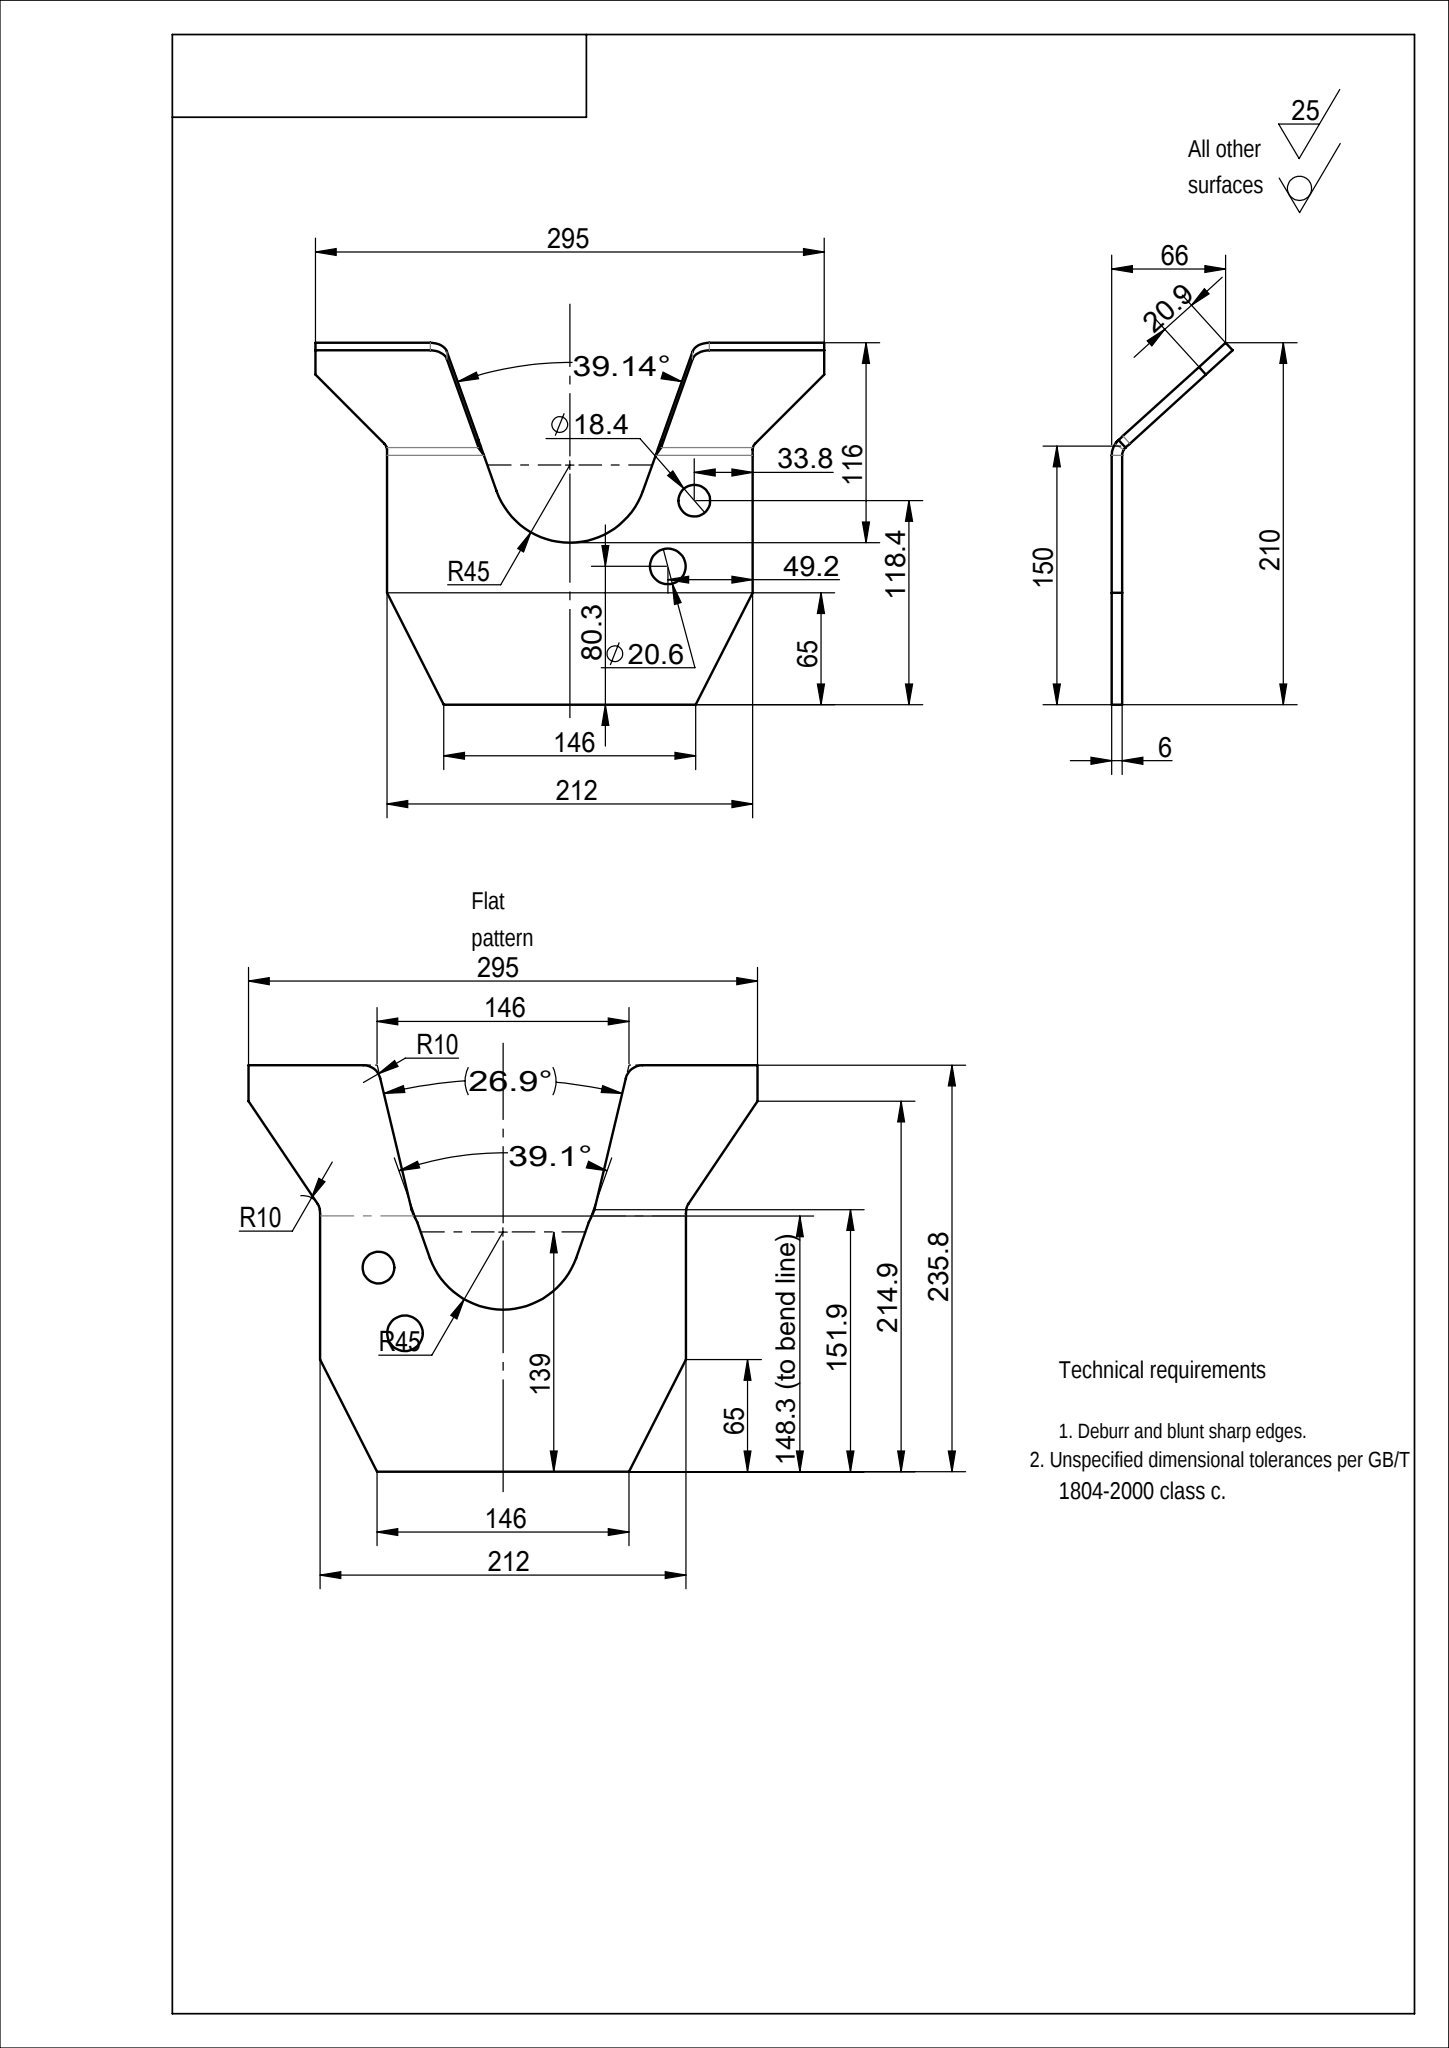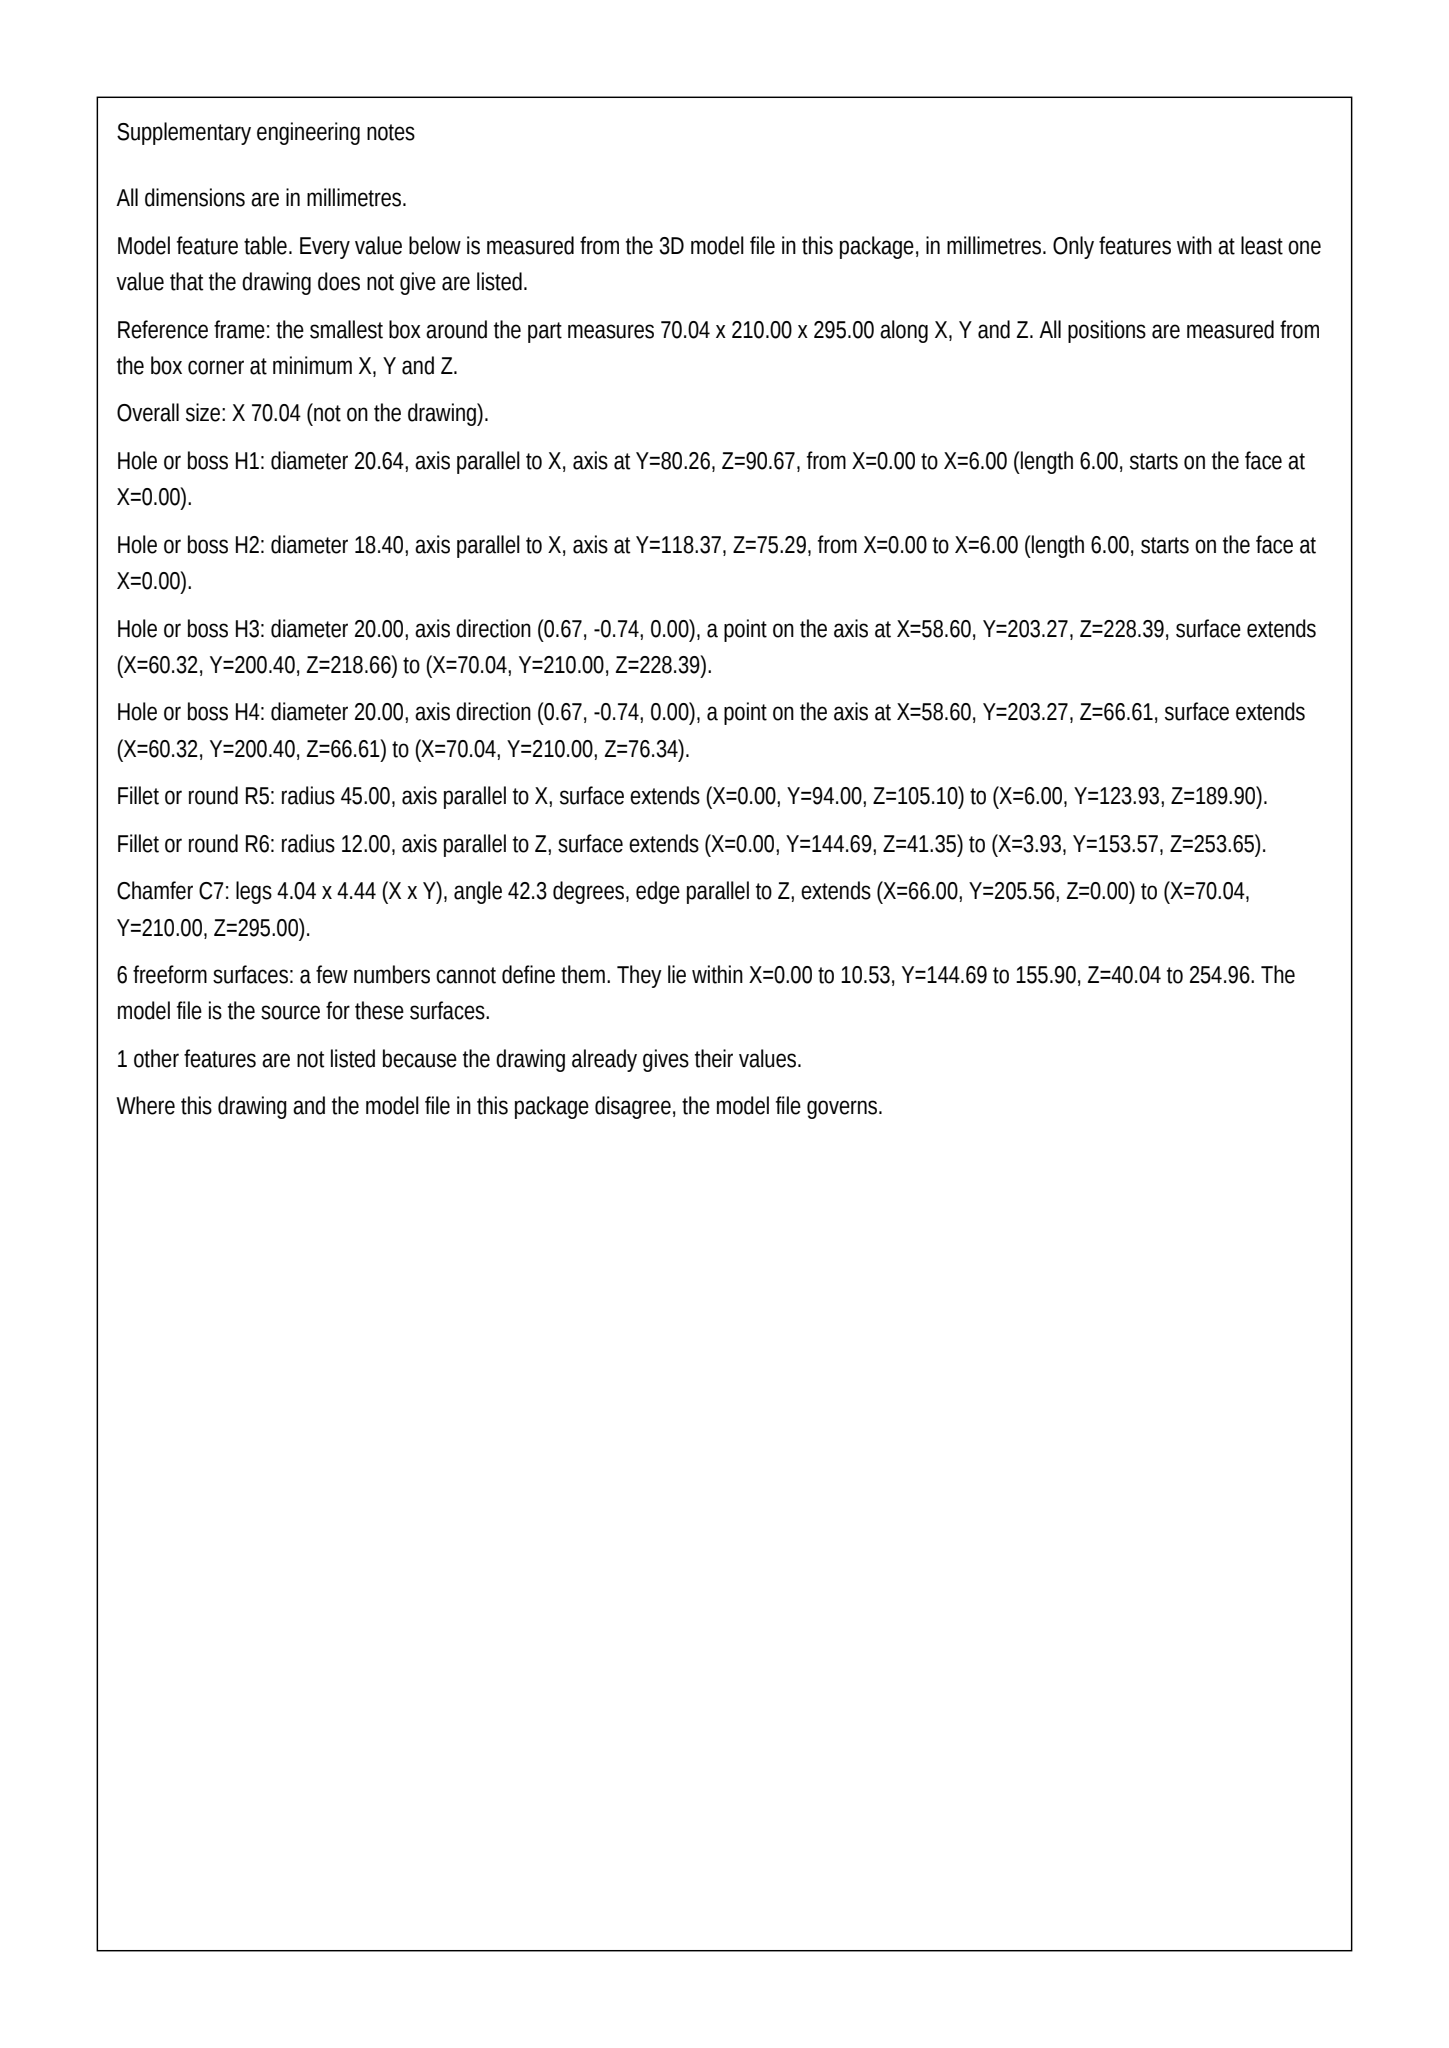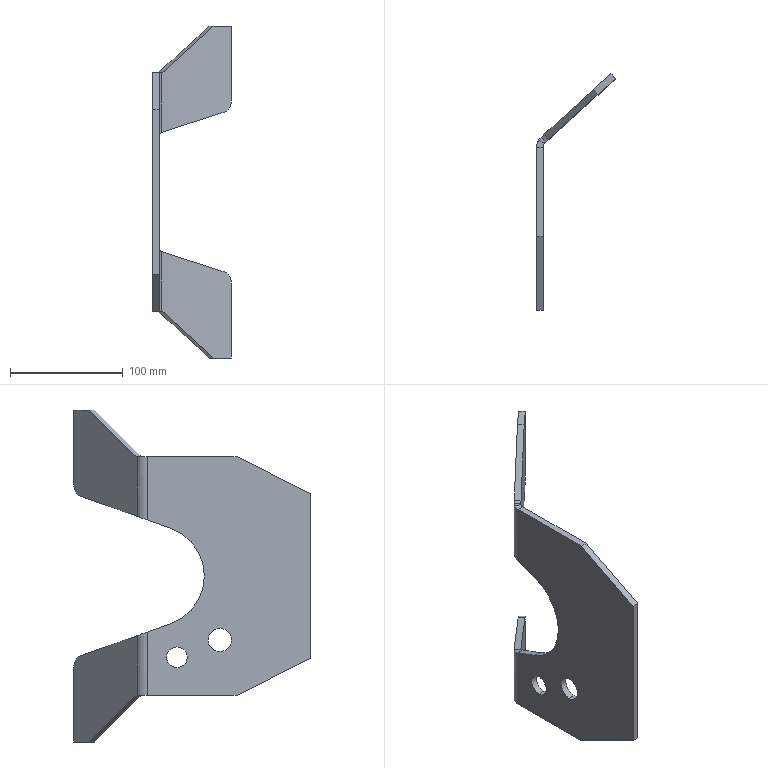Part | SolidWorks | mm | 1 solid | 40 faces | box 70.04 x 210 x 295 mm | volume 218850 mm3 | plane 23 | cylinder 11 | spline 6 | commonest cylinder face diameters 20.64 x2 20 x2 24 x2 12 x2 18.395 x2 90 x1